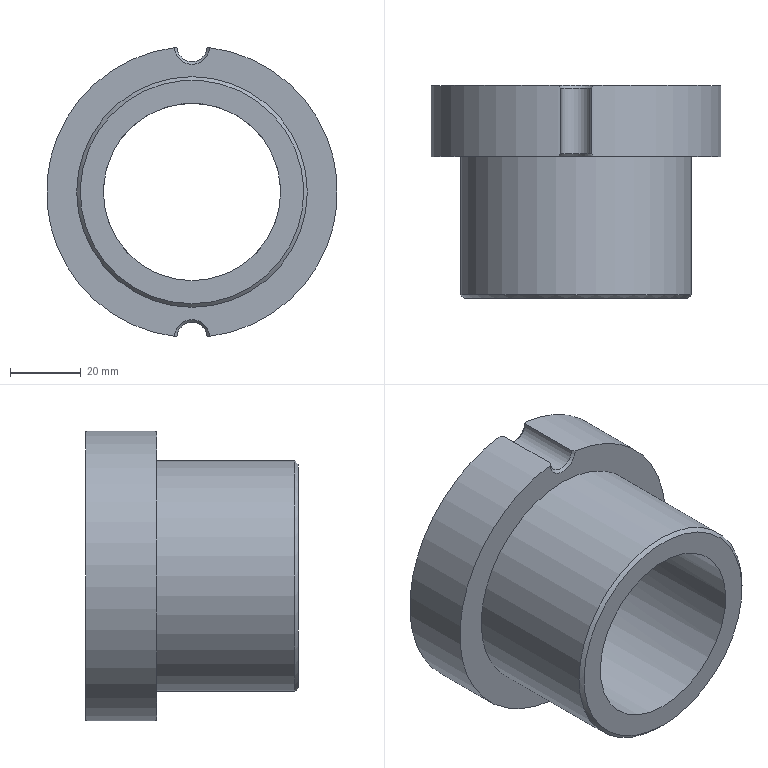Component | NX | NUT | 1 solid | 15 faces | volume 117993 mm3 | cylinder 6 | cone 6 | plane 3 | commonest cylinder face diameters 82 x2 8.5 x2 65 x1 50 x1